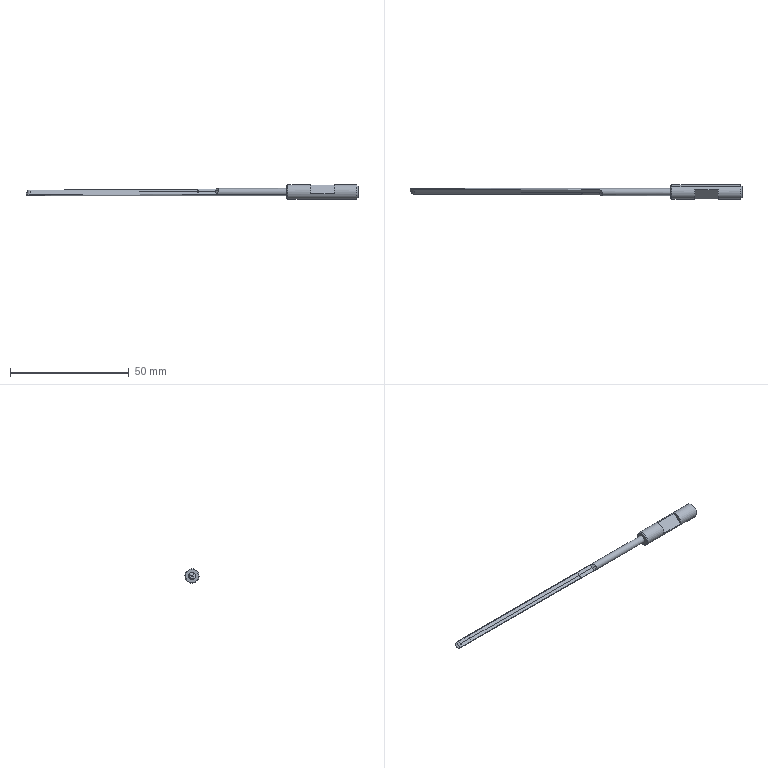Component | SolidWorks | JJDJR-3060-E-025-1 | 1 solid | 32 faces | volume 1272 mm3 | plane 17 | cylinder 8 | cone 5 | spline 2 | commonest cylinder face diameters 0.3 x3 3 x2 6 x2 4 x1 | material Aluminum Alloy